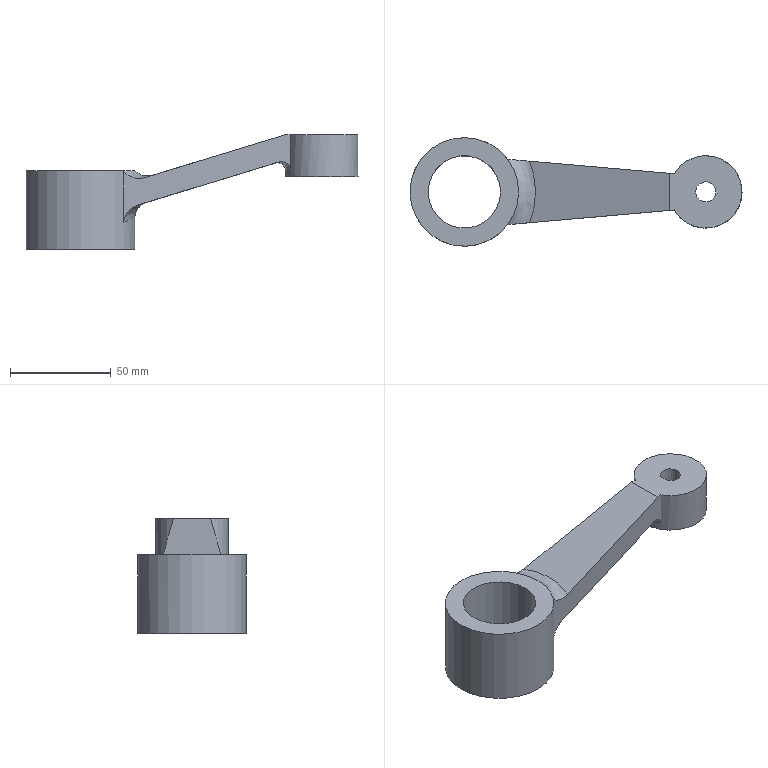Component | NX | PART_DRAWING | 1 solid | 15 faces | volume 94564 mm3 | plane 8 | cylinder 4 | spline 3 | commonest cylinder face diameters 36 x2 10 x1 54 x1